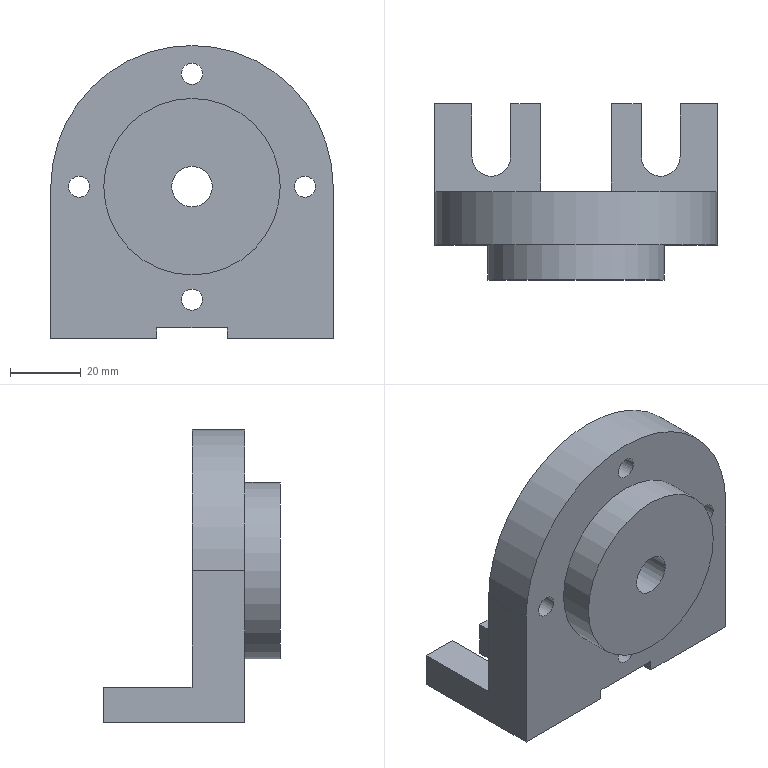Component | NX | REAR_COVER | 1 solid | 38 faces | volume 111605 mm3 | plane 24 | cylinder 13 | cone 1 | commonest cylinder face diameters 6 x4 12 x4 11 x2 80 x1 50 x1 11.5 x1